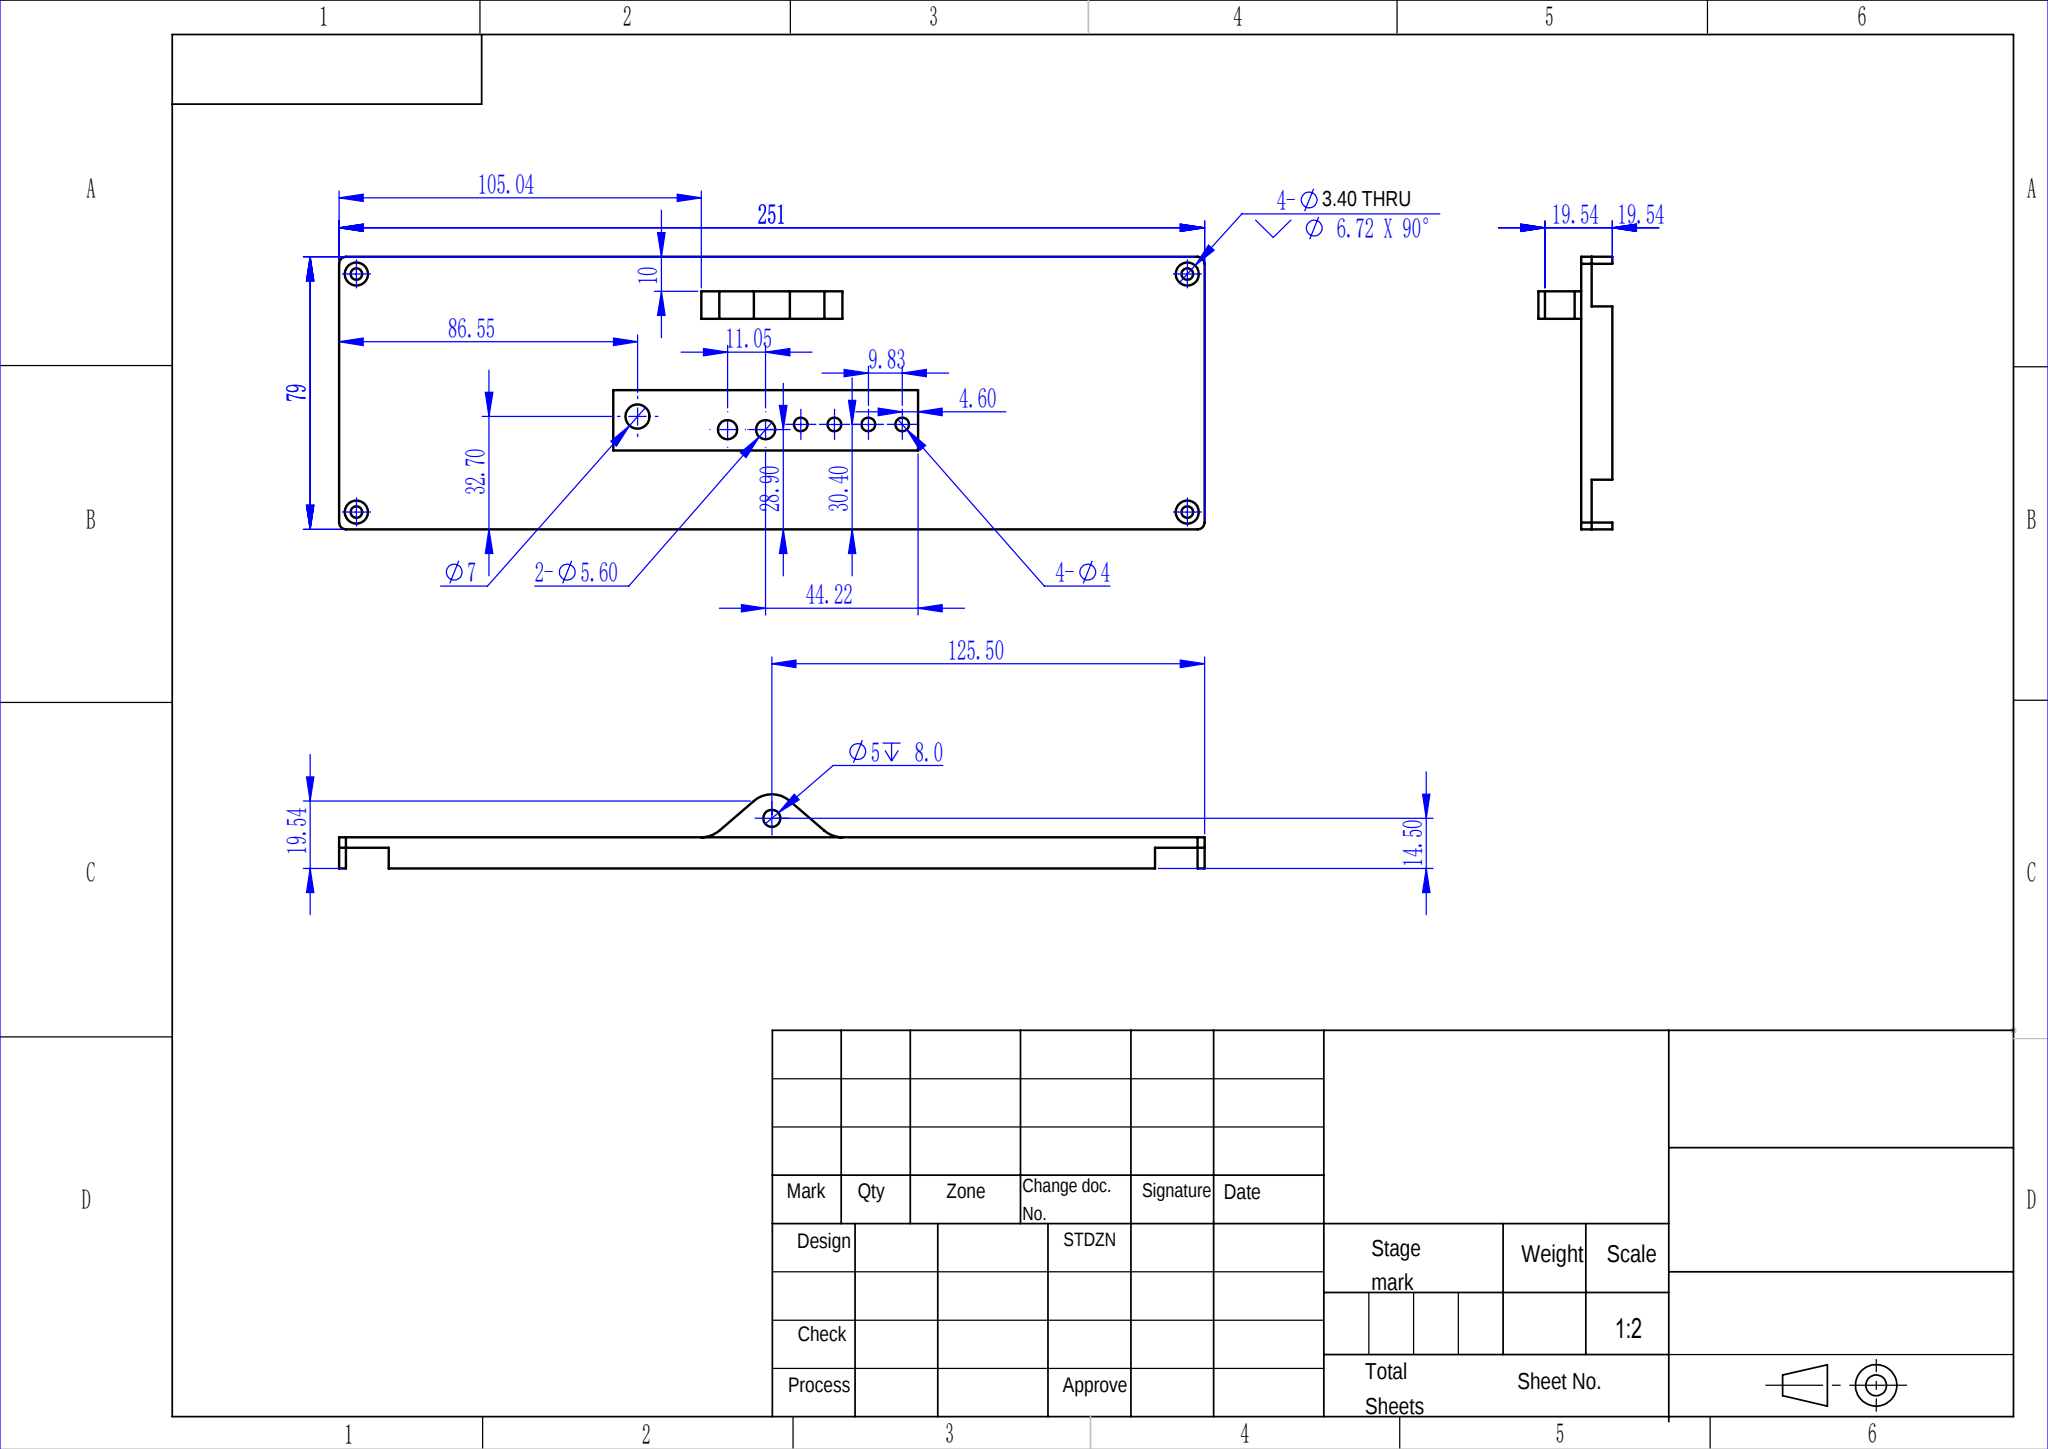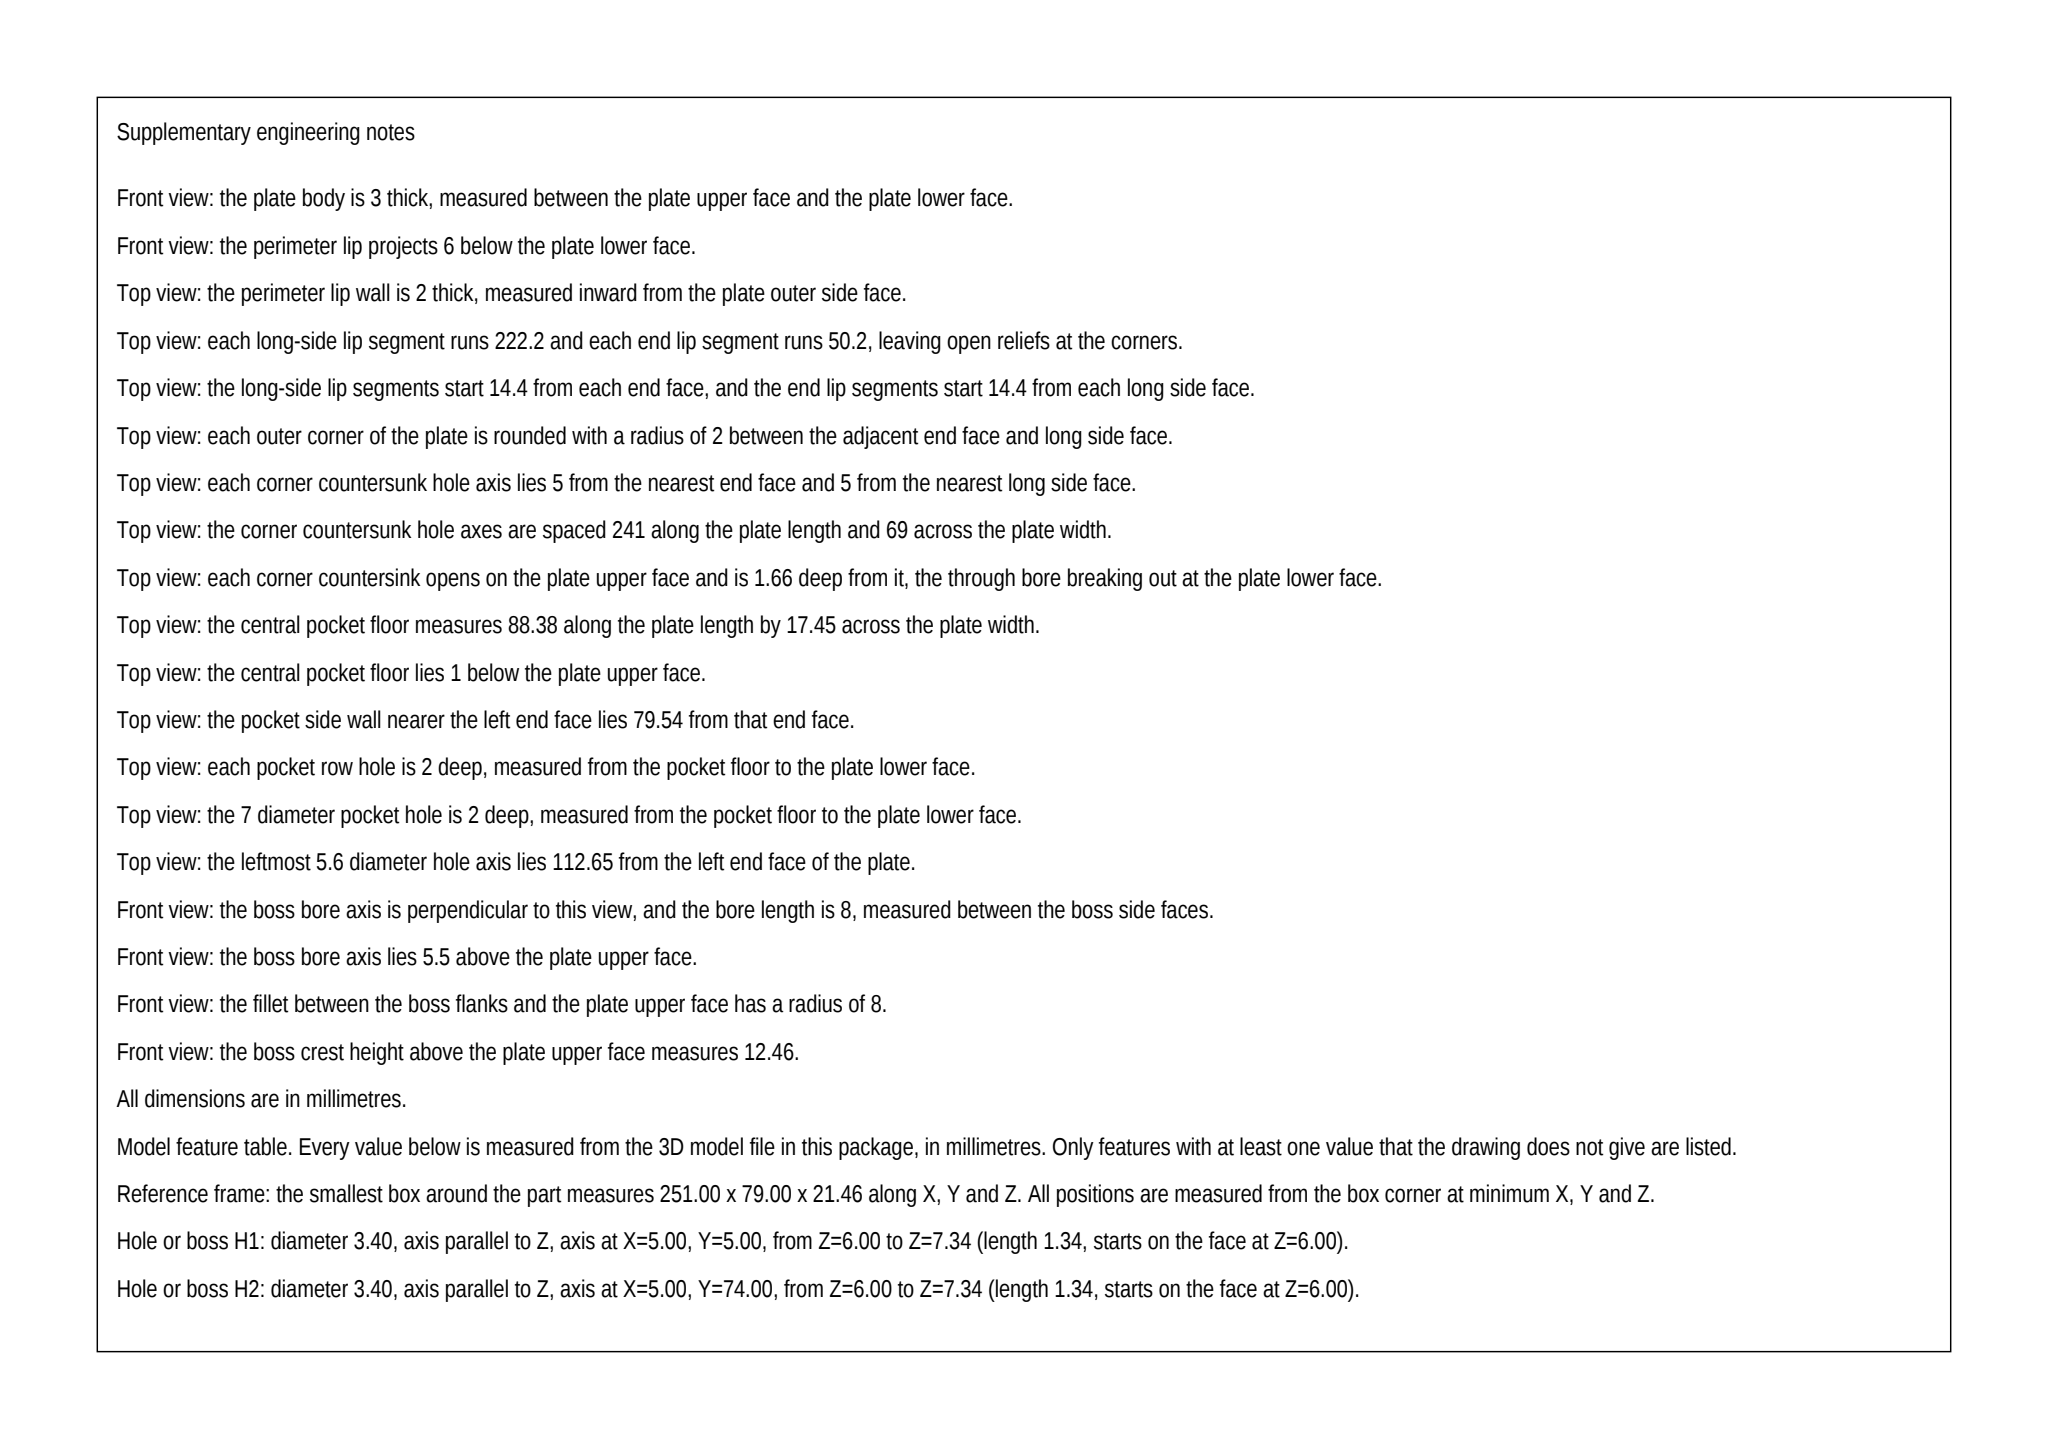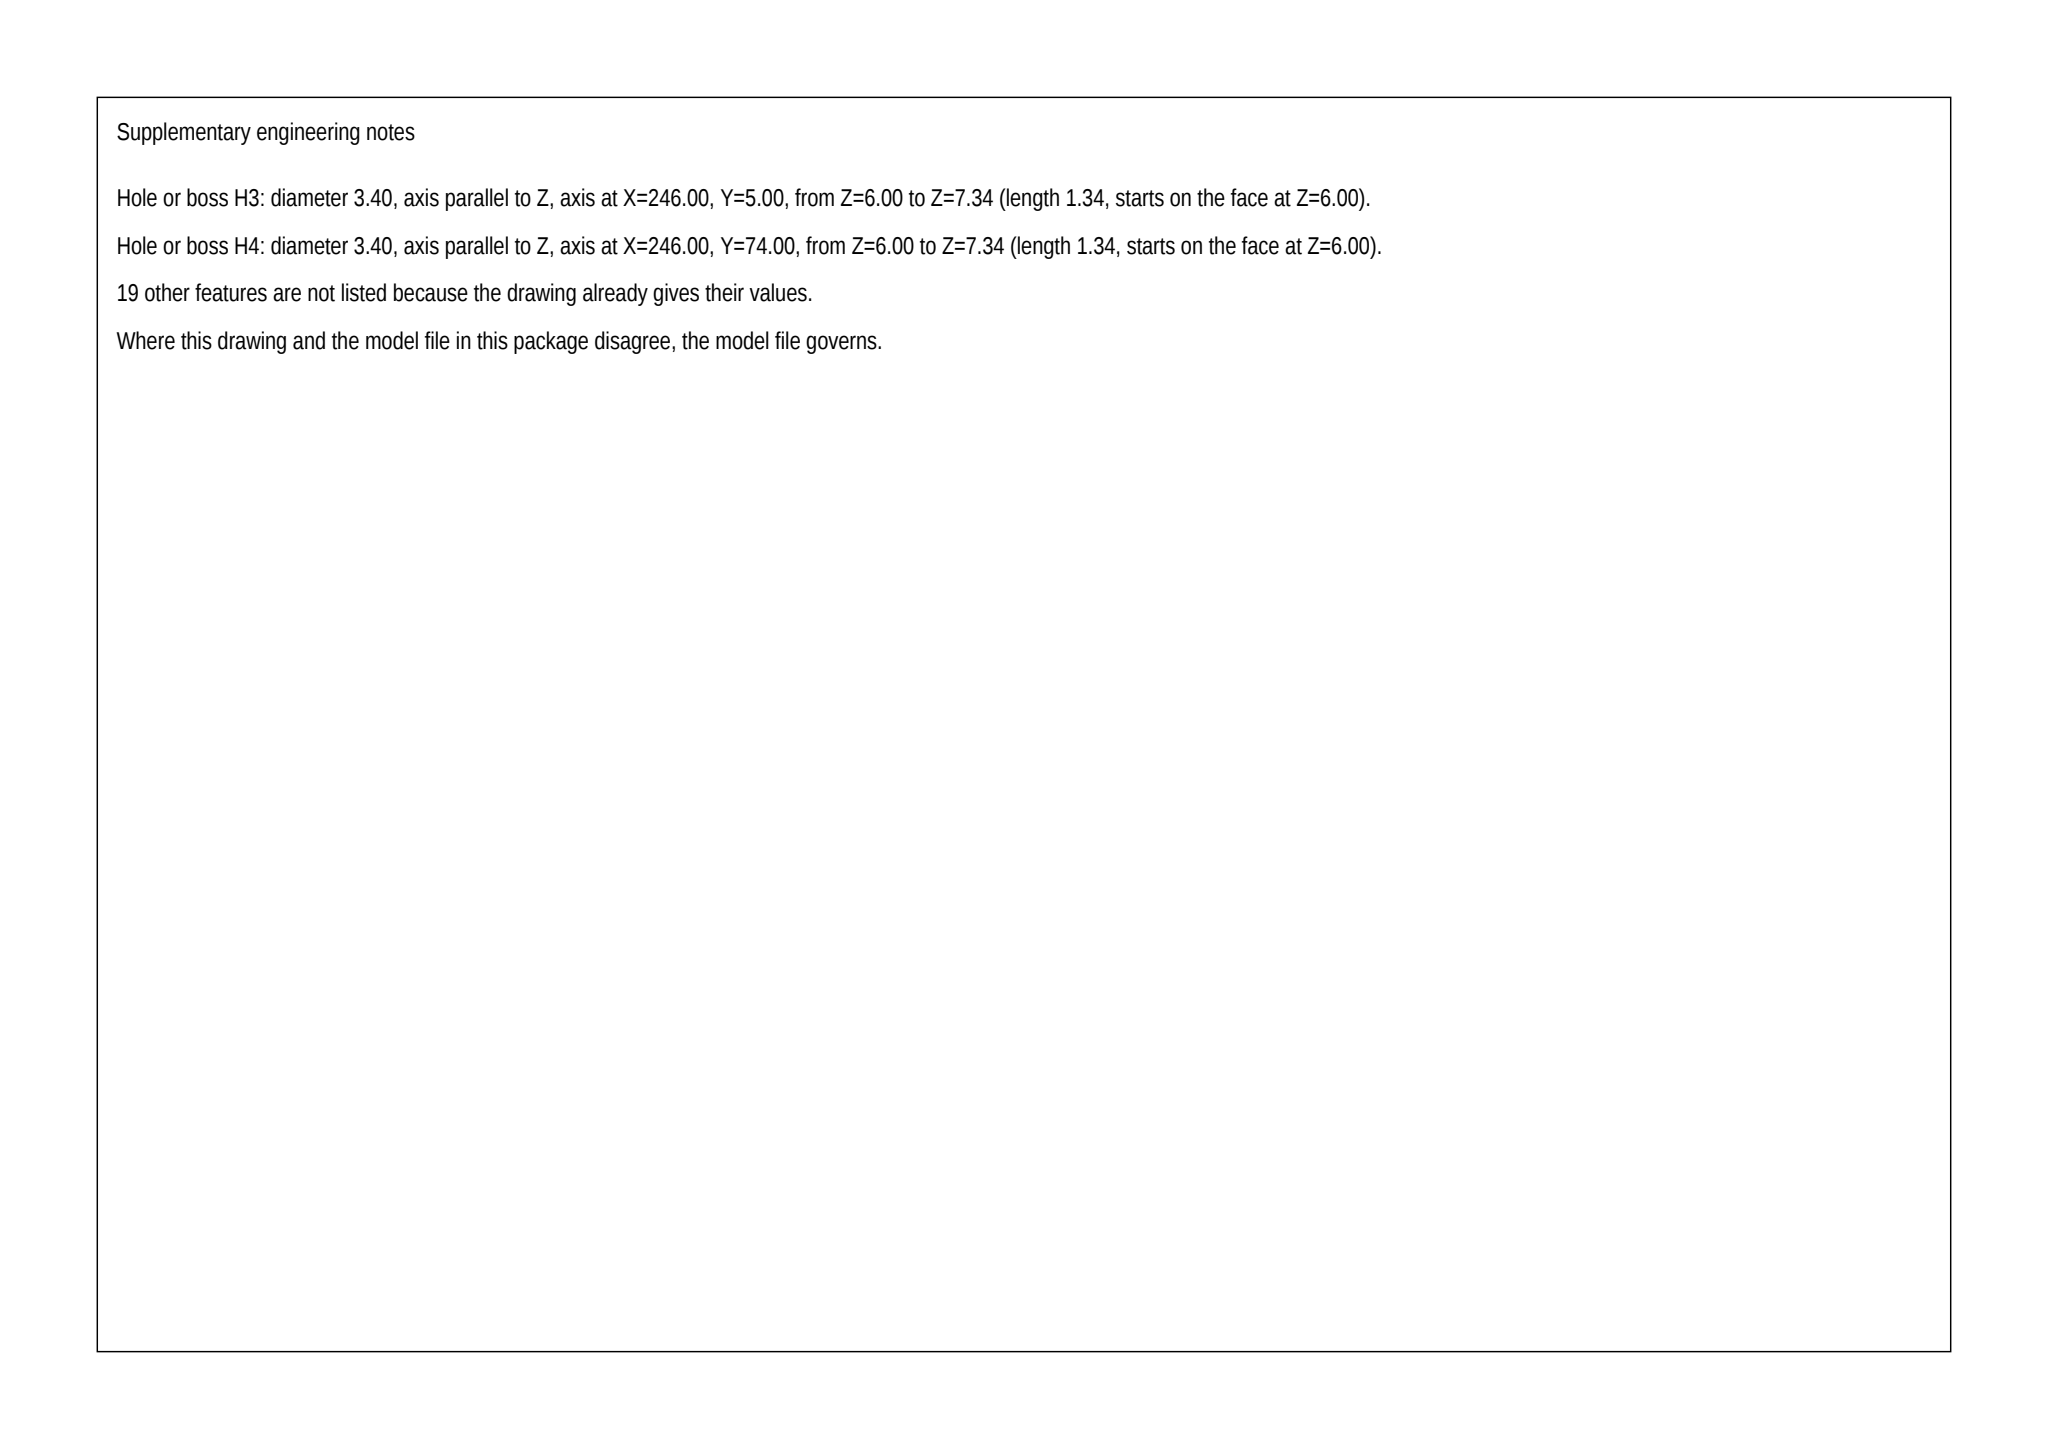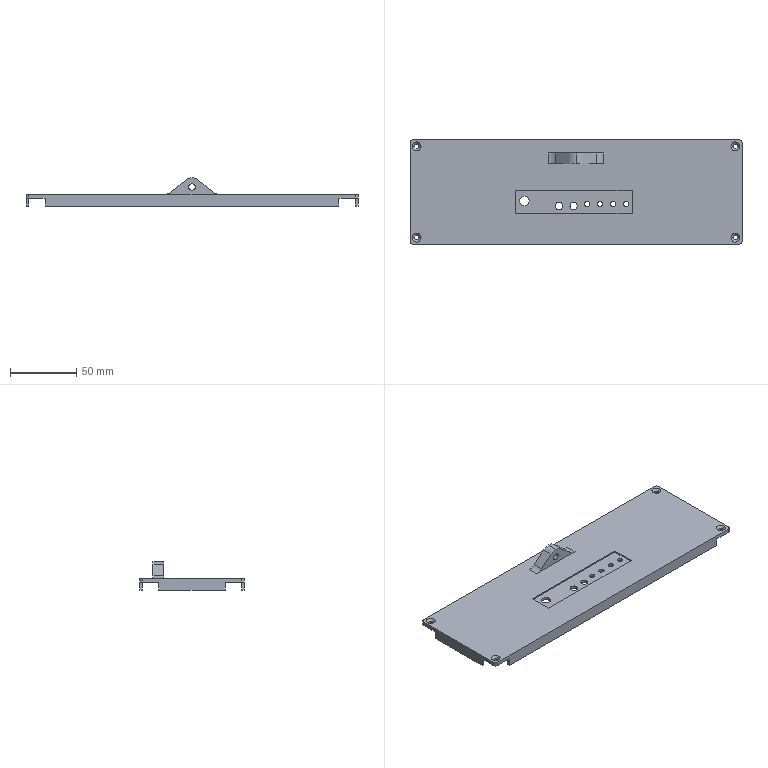Part | SolidWorks | mm | 1 solid | 71 faces | box 251 x 79 x 21.46 mm | volume 65892 mm3 | cylinder 32 | plane 31 | cone 8 | commonest cylinder face diameters 4 x12 3.4 x8 16 x4 5.6 x4 5 x2 7 x2
Drawing notes:
OVERALL 251 X 79 X 21.46 HIGH | from the solid: bbox_xyz 251.0 x 79.0 x 21.463
FROM BTM FACE: STEPS AT 6 & 8, PLATE TOP 9, RIB TOP 21.46 | from the solid: z planes 0 (datum), 6, 8, 9; bbox z max 21.463
STEP FACE 14.40 IN FROM EACH EDGE, 4 SIDES | from the solid: x planes 14.4 & 236.6 (251-14.4); y planes 14.4 & 64.6 (79-14.4), 2 faces each
CTR RIB 40.92 LG X 8 WIDE, 105.04 FROM LH EDGE, 10 FROM TOP EDGE, TOP AT 21.46 | from the solid: Y-axis Ø16 cyls x=105.04/125.50/145.96 (R8 blends), 8 lg; y planes 61.0 & 69.0 (79-69=10); bbox z 21.463
2-Ø5.60 ON CL 28.90 FROM BTM EDGE, AT 112.65 & 123.70 FROM LH EDGE | from the solid: Ø5.6 z-holes y=28.9 at x=112.65 and 123.70, 2.0 DP
4-Ø4 ROW ON CL 30.40, 1ST HOLE 133.88 FROM LH EDGE, SP 9.77/9.84/9.83 | from the solid: Ø4 z-holes y=30.4 at x=133.88, 143.65, 153.49, 163.32 (29.44 overall)
Ø7 DP 2 | from the solid: cylinder dia 7, axis z at (86.55,32.70), length 2.0
2-Ø5.60 DP 2 | from the solid: cylinders dia 5.6, axis z at (112.65,28.9) and (123.70,28.9), length 2.0
4-Ø4 DP 2 | from the solid: cylinders dia 4, axis z at x=133.88/143.65/153.49/163.32, y=30.4, length 2.0